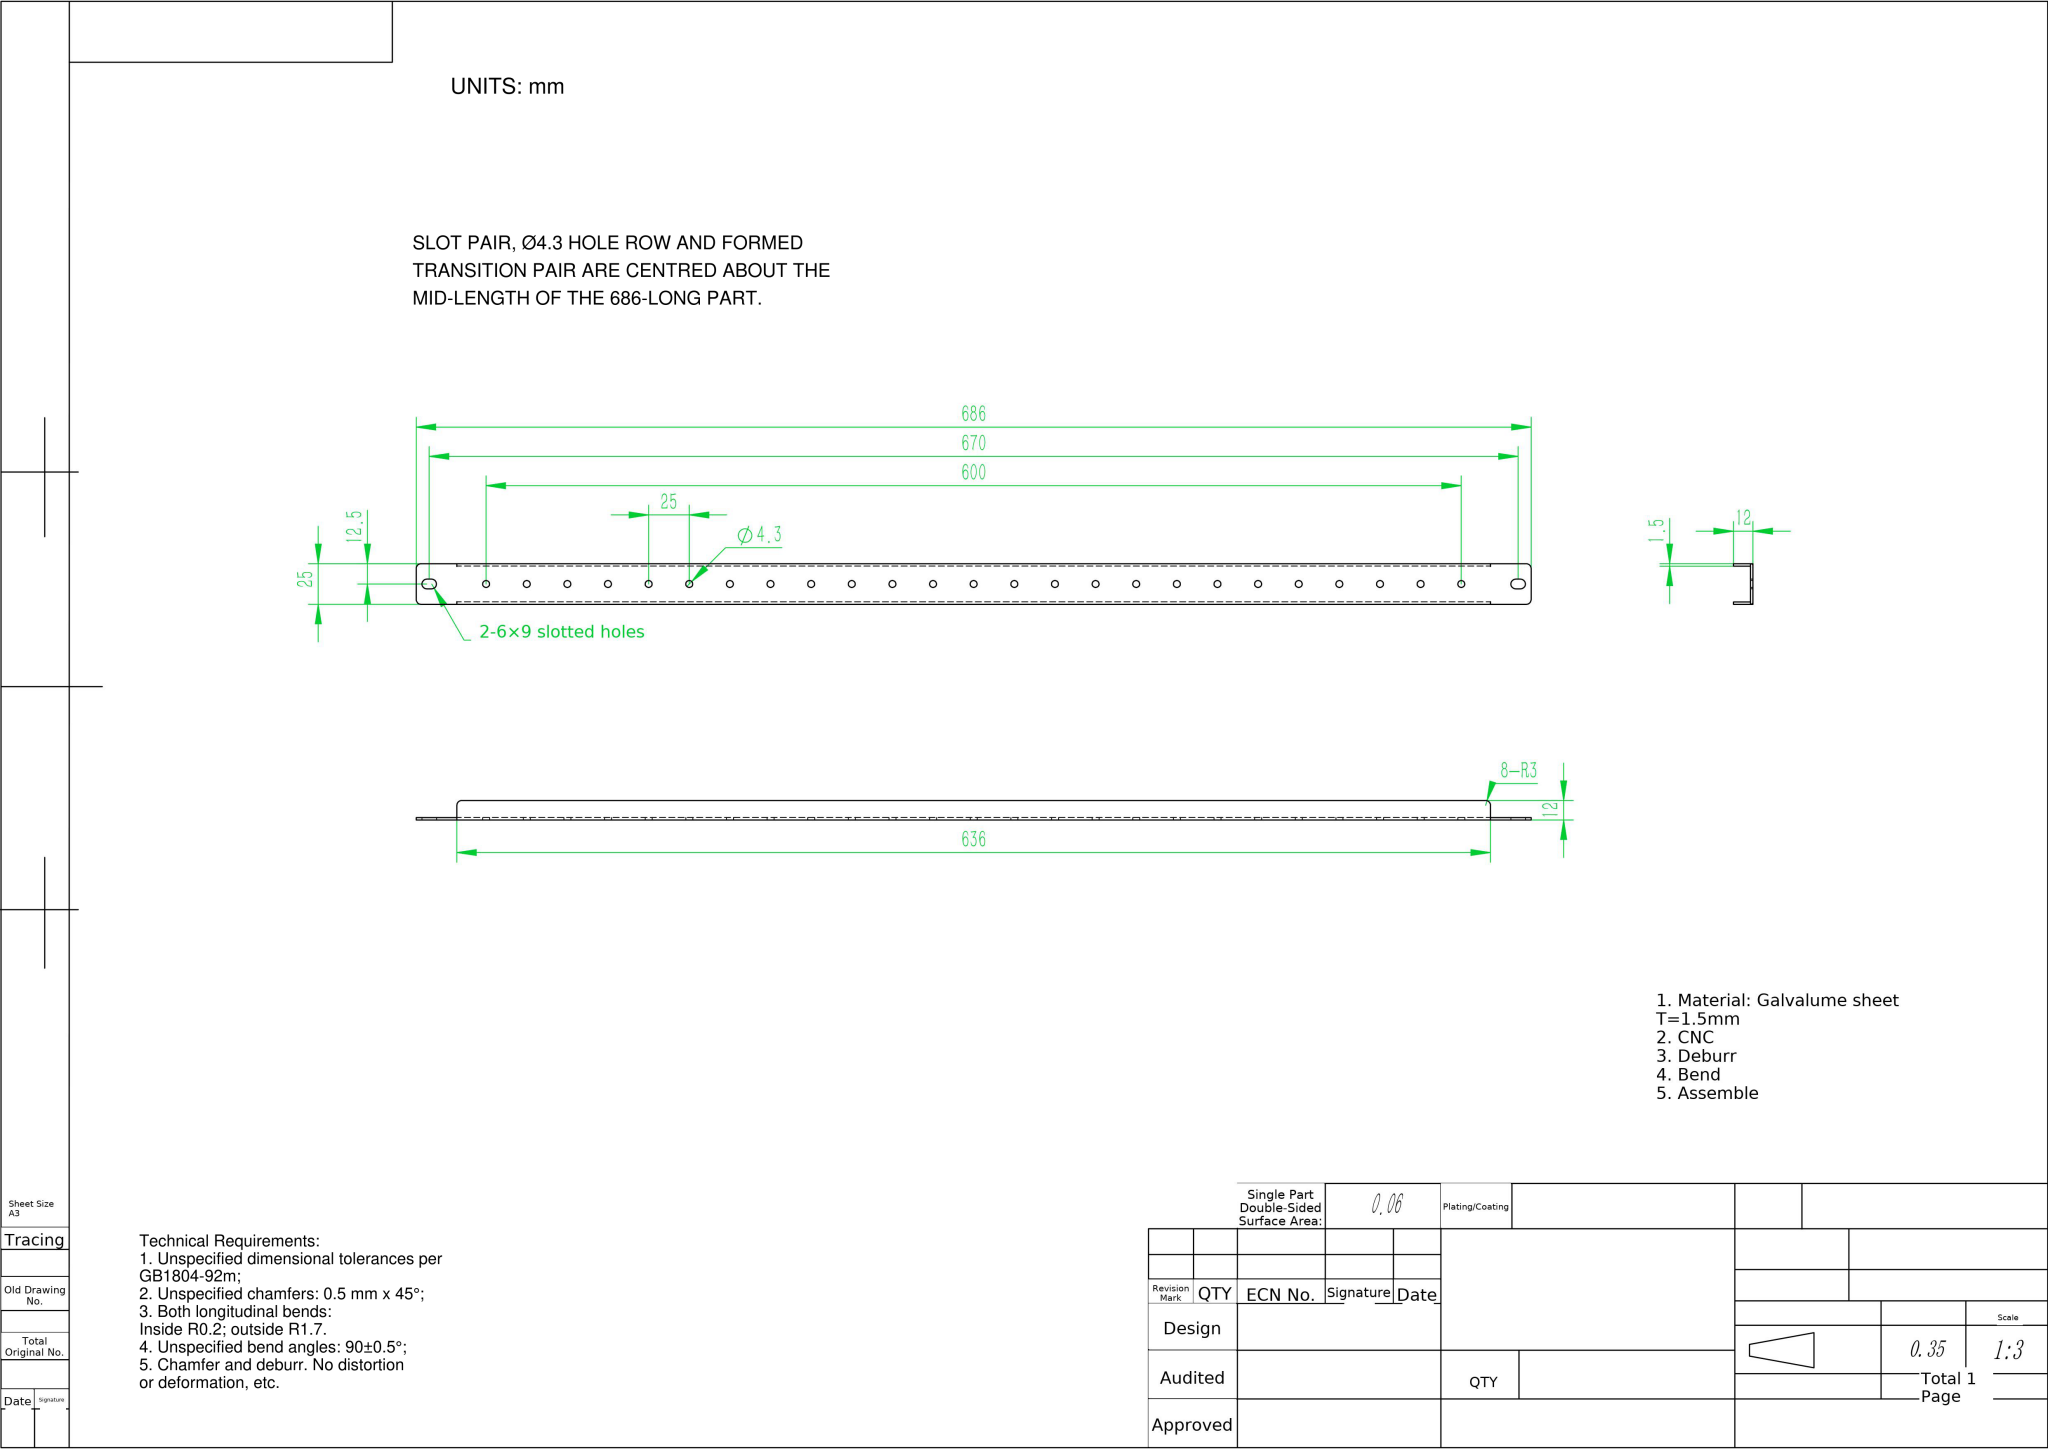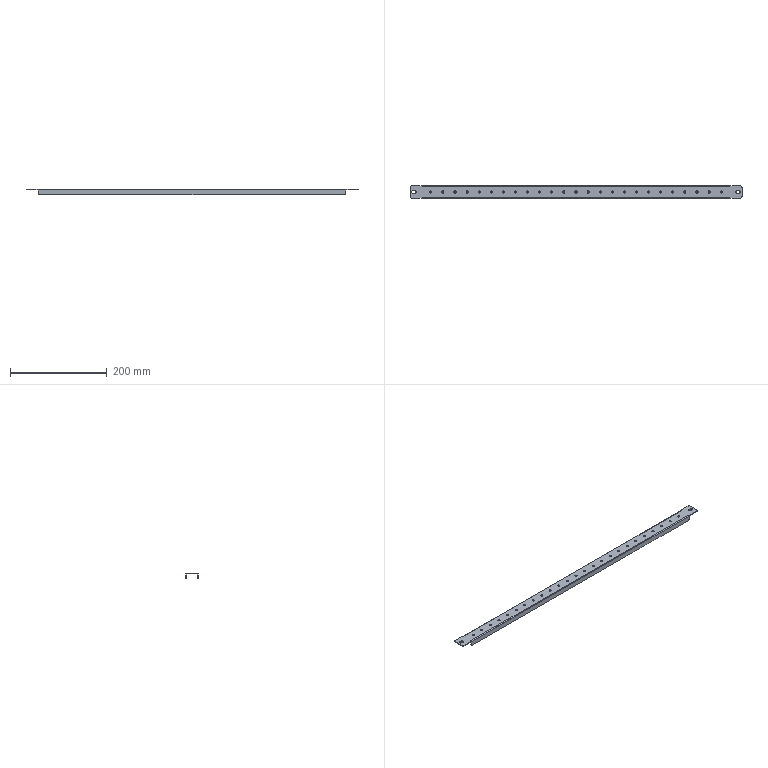Part | NX | mm | 1 solid | 98 faces | box 686 x 25 x 12 mm | volume 44274 mm3 | cylinder 68 | plane 30 | commonest cylinder face diameters 4.3 x50 6 x14 3.4 x2 0.4 x2